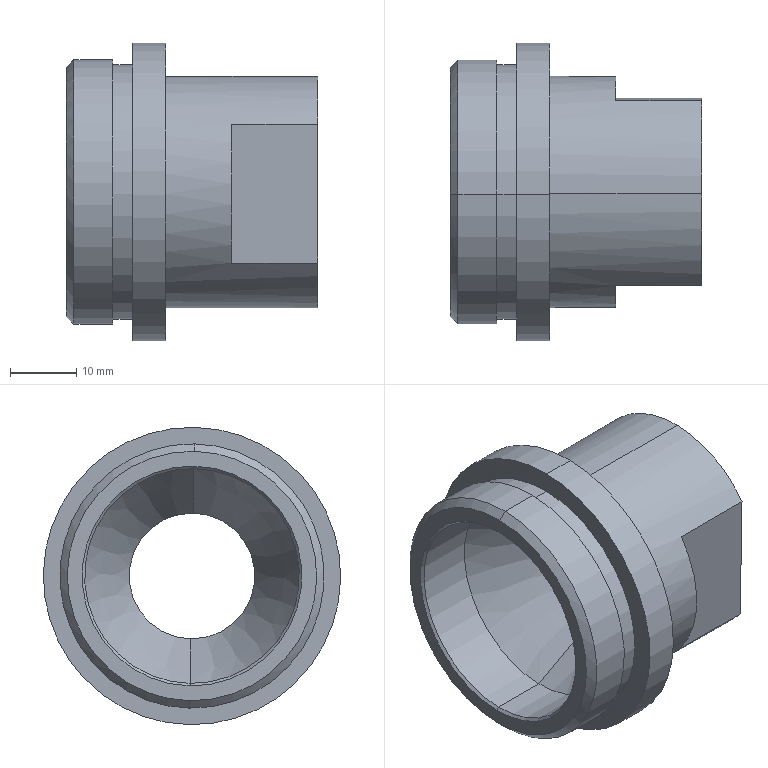Component | SolidWorks | 216InnerTubeAssembly-1_ValveGland-1 | 1 solid | 27 faces | box 38 x 45 x 45 mm | volume 22275 mm3 | cylinder 12 | plane 9 | cone 6 | commonest cylinder face diameters 40 x2 38.502 x2 45 x2 35 x2 19.03 x2 32.511 x2 | material Alloy Steel
build123d program:
from build123d import *

# Parameters (mm, degrees)
CUT_EXTRUDE1_DEPTH = 13


with BuildPart() as part:
    # Model → Revolve1 (revolve)
    with BuildSketch(Plane.XY, mode=Mode.PRIVATE) as revolve1_sk:
        Polygon((-37.447, 16.234), (-37.821, 16.608), (-37.821, 18.855), (-36.698, 19.979), (-30.821, 19.979), (-30.821, 19.23), (-27.821, 19.23), (-27.821, 22.479), (-22.821, 22.479), (-22.821, 17.479), (0.1786, 17.479), (0.1786, 9.494), (-16.821, 9.494), (-28.821, 16.234), align=None)
    revolve(revolve1_sk.sketch.rotate(Axis((1.198, -0.02131, 0), (-1, 0, 0)), 90), axis=Axis((1.198, -0.02131, 0), (-1, 0, 0)))

    # Sketch2 → Cut-Extrude1 (cut)
    with BuildSketch(Plane(origin=(0.1786, 0, 0), x_dir=(0, 0, -1), z_dir=(1, 0, 0))):
        with BuildLine():
            Line((-14.873, 13.979), (14.873, 13.979))
            ThreePointArc((14.873, 13.979), (0, 20.404), (-14.873, 13.979))
        make_face()
        with BuildLine():
            Line((-14.873, -14.021), (14.873, -14.021))
            ThreePointArc((14.873, -14.021), (0, -20.447), (-14.873, -14.021))
        make_face()
    extrude(amount=-CUT_EXTRUDE1_DEPTH, mode=Mode.SUBTRACT)


solid = part.part

# Placed as in the assembly
solid = solid.moved(Location((1191.249, 0.02131, 0.0003826), (1.029, 0, 0)))
STEP:
#1=COLOUR_RGB('',0.7922,0.8196,0.9333);
#2=FILL_AREA_STYLE_COLOUR('',#1);
#3=FILL_AREA_STYLE('',(#2));
#4=SURFACE_STYLE_FILL_AREA(#3);
#5=SURFACE_SIDE_STYLE('',(#4));
#6=SURFACE_STYLE_USAGE(.BOTH.,#5);
#7=PRESENTATION_STYLE_ASSIGNMENT((#6));
#8=CARTESIAN_POINT('',(45.425,-0.01149,0.6399));
#9=VERTEX_POINT('',#8);
#10=CARTESIAN_POINT('',(45.425,0.01149,-0.6399));
#11=VERTEX_POINT('',#10);
#12=CARTESIAN_POINT('',(45.425,-0.,0.));
#13=DIRECTION('',(1.,0.,-0.));
#14=DIRECTION('',(0.,0.01796,-0.9998));
#15=AXIS2_PLACEMENT_3D('',#12,#13,#14);
#16=CIRCLE('',#15,0.64);
#17=EDGE_CURVE('',#9,#11,#16,.T.);
#18=ORIENTED_EDGE('',*,*,#17,.T.);
#19=CARTESIAN_POINT('',(45.411,0.01176,-0.6546));
#20=VERTEX_POINT('',#19);
#21=CARTESIAN_POINT('',(45.411,0.01176,-0.6546));
#22=DIRECTION('',(-0.7071,0.0127,-0.707));
#23=VECTOR('',#22,39.37);
#24=LINE('',#21,#23);
#25=EDGE_CURVE('',#11,#20,#24,.T.);
#26=ORIENTED_EDGE('',*,*,#25,.T.);
#27=CARTESIAN_POINT('',(45.411,-0.01176,0.6546));
#28=VERTEX_POINT('',#27);
#29=CARTESIAN_POINT('',(45.411,-0.,0.));
#30=DIRECTION('',(1.,0.,-0.));
#31=DIRECTION('',(0.,0.01796,-0.9998));
#32=AXIS2_PLACEMENT_3D('',#29,#30,#31);
#33=CIRCLE('',#32,0.6547);
#34=EDGE_CURVE('',#28,#20,#33,.T.);
#35=ORIENTED_EDGE('',*,*,#34,.F.);
#36=CARTESIAN_POINT('',(45.411,-0.01176,0.6546));
#37=DIRECTION('',(-0.7071,-0.0127,0.707));
#38=VECTOR('',#37,39.37);
#39=LINE('',#36,#38);
#40=EDGE_CURVE('',#9,#28,#39,.T.);
#41=ORIENTED_EDGE('',*,*,#40,.F.);
#42=EDGE_LOOP('',(#18,#26,#35,#41));
#43=FACE_OUTER_BOUND('',#42,.T.);
#44=CARTESIAN_POINT('',(45.411,-0.,0.));
#45=DIRECTION('',(-1.,-0.,0.));
#46=DIRECTION('',(0.,-0.01796,0.9998));
#47=AXIS2_PLACEMENT_3D('',#44,#45,#46);
#48=CONICAL_SURFACE('',#47,0.6547,0.7854);
#49=ADVANCED_FACE('',(#43),#48,.F.);
#50=CARTESIAN_POINT('',(45.411,0.01334,-0.7431));
#51=VERTEX_POINT('',#50);
#52=CARTESIAN_POINT('',(45.411,-0.01334,0.7431));
#53=VERTEX_POINT('',#52);
#54=CARTESIAN_POINT('',(45.411,-0.,0.));
#55=DIRECTION('',(1.,0.,-0.));
#56=DIRECTION('',(0.,0.01796,-0.9998));
#57=AXIS2_PLACEMENT_3D('',#54,#55,#56);
#58=CIRCLE('',#57,0.7432);
#59=EDGE_CURVE('',#51,#53,#58,.T.);
#60=ORIENTED_EDGE('',*,*,#59,.T.);
#61=CARTESIAN_POINT('',(45.455,-0.01414,0.7873));
#62=VERTEX_POINT('',#61);
#63=CARTESIAN_POINT('',(45.455,-0.01414,0.7873));
#64=DIRECTION('',(0.7071,-0.0127,0.707));
#65=VECTOR('',#64,39.37);
#66=LINE('',#63,#65);
#67=EDGE_CURVE('',#53,#62,#66,.T.);
#68=ORIENTED_EDGE('',*,*,#67,.T.);
#69=CARTESIAN_POINT('',(45.455,0.01414,-0.7873));
#70=VERTEX_POINT('',#69);
#71=CARTESIAN_POINT('',(45.455,-0.,0.));
#72=DIRECTION('',(1.,0.,-0.));
#73=DIRECTION('',(0.,0.01796,-0.9998));
#74=AXIS2_PLACEMENT_3D('',#71,#72,#73);
#75=CIRCLE('',#74,0.7874);
#76=EDGE_CURVE('',#70,#62,#75,.T.);
#77=ORIENTED_EDGE('',*,*,#76,.F.);
#78=CARTESIAN_POINT('',(45.455,0.01414,-0.7873));
#79=DIRECTION('',(0.7071,0.0127,-0.707));
#80=VECTOR('',#79,39.37);
#81=LINE('',#78,#80);
#82=EDGE_CURVE('',#51,#70,#81,.T.);
#83=ORIENTED_EDGE('',*,*,#82,.F.);
#84=EDGE_LOOP('',(#60,#68,#77,#83));
#85=FACE_OUTER_BOUND('',#84,.T.);
#86=CARTESIAN_POINT('',(45.455,-0.,0.));
#87=DIRECTION('',(1.,0.,-0.));
#88=DIRECTION('',(0.,0.01796,-0.9998));
#89=AXIS2_PLACEMENT_3D('',#86,#87,#88);
#90=CONICAL_SURFACE('',#89,0.7874,0.7854);
#91=ADVANCED_FACE('',(#85),#90,.T.);
#92=ORIENTED_EDGE('',*,*,#76,.T.);
#93=CARTESIAN_POINT('',(45.686,-0.01414,0.7873));
#94=VERTEX_POINT('',#93);
#95=CARTESIAN_POINT('',(46.947,-0.01414,0.7873));
#96=DIRECTION('',(1.,0.,-0.));
#97=VECTOR('',#96,39.37);
#98=LINE('',#95,#97);
#99=EDGE_CURVE('',#62,#94,#98,.T.);
#100=ORIENTED_EDGE('',*,*,#99,.T.);
#101=CARTESIAN_POINT('',(45.686,0.01414,-0.7873));
#102=VERTEX_POINT('',#101);
#103=CARTESIAN_POINT('',(45.686,-0.,0.));
#104=DIRECTION('',(1.,0.,-0.));
#105=DIRECTION('',(0.,0.01796,-0.9998));
#106=AXIS2_PLACEMENT_3D('',#103,#104,#105);
#107=CIRCLE('',#106,0.7874);
#108=EDGE_CURVE('',#102,#94,#107,.T.);
#109=ORIENTED_EDGE('',*,*,#108,.F.);
#110=CARTESIAN_POINT('',(46.947,0.01414,-0.7873));
#111=DIRECTION('',(1.,0.,-0.));
#112=VECTOR('',#111,39.37);
#113=LINE('',#110,#112);
#114=EDGE_CURVE('',#70,#102,#113,.T.);
#115=ORIENTED_EDGE('',*,*,#114,.F.);
#116=EDGE_LOOP('',(#92,#100,#109,#115));
#117=FACE_OUTER_BOUND('',#116,.T.);
#118=CARTESIAN_POINT('',(46.947,-0.,0.));
#119=DIRECTION('',(1.,0.,-0.));
#120=DIRECTION('',(0.,0.01796,-0.9998));
#121=AXIS2_PLACEMENT_3D('',#118,#119,#120);
#122=CYLINDRICAL_SURFACE('',#121,0.7874);
#123=ADVANCED_FACE('',(#117),#122,.T.);
#124=CARTESIAN_POINT('',(45.686,0.01361,-0.7578));
#125=VERTEX_POINT('',#124);
#126=CARTESIAN_POINT('',(45.686,-0.01361,0.7578));
#127=VERTEX_POINT('',#126);
#128=CARTESIAN_POINT('',(45.686,-0.,0.));
#129=DIRECTION('',(1.,0.,-0.));
#130=DIRECTION('',(0.,0.01796,-0.9998));
#131=AXIS2_PLACEMENT_3D('',#128,#129,#130);
#132=CIRCLE('',#131,0.7579);
#133=EDGE_CURVE('',#125,#127,#132,.T.);
#134=ORIENTED_EDGE('',*,*,#133,.T.);
#135=CARTESIAN_POINT('',(45.804,-0.01361,0.7578));
#136=VERTEX_POINT('',#135);
#137=CARTESIAN_POINT('',(46.947,-0.01361,0.7578));
#138=DIRECTION('',(1.,0.,-0.));
#139=VECTOR('',#138,39.37);
#140=LINE('',#137,#139);
#141=EDGE_CURVE('',#127,#136,#140,.T.);
#142=ORIENTED_EDGE('',*,*,#141,.T.);
#143=CARTESIAN_POINT('',(45.804,0.01361,-0.7578));
#144=VERTEX_POINT('',#143);
#145=CARTESIAN_POINT('',(45.804,-0.,0.));
#146=DIRECTION('',(1.,0.,-0.));
#147=DIRECTION('',(0.,0.01796,-0.9998));
#148=AXIS2_PLACEMENT_3D('',#145,#146,#147);
#149=CIRCLE('',#148,0.7579);
#150=EDGE_CURVE('',#144,#136,#149,.T.);
#151=ORIENTED_EDGE('',*,*,#150,.F.);
#152=CARTESIAN_POINT('',(46.947,0.01361,-0.7578));
#153=DIRECTION('',(1.,0.,-0.));
#154=VECTOR('',#153,39.37);
#155=LINE('',#152,#154);
#156=EDGE_CURVE('',#125,#144,#155,.T.);
#157=ORIENTED_EDGE('',*,*,#156,.F.);
#158=EDGE_LOOP('',(#134,#142,#151,#157));
#159=FACE_OUTER_BOUND('',#158,.T.);
#160=CARTESIAN_POINT('',(46.947,-0.,0.));
#161=DIRECTION('',(1.,0.,-0.));
#162=DIRECTION('',(0.,0.01796,-0.9998));
#163=AXIS2_PLACEMENT_3D('',#160,#161,#162);
#164=CYLINDRICAL_SURFACE('',#163,0.7579);
#165=ADVANCED_FACE('',(#159),#164,.T.);
#166=CARTESIAN_POINT('',(45.804,0.01591,-0.8857));
#167=VERTEX_POINT('',#166);
#168=CARTESIAN_POINT('',(45.804,-0.01591,0.8857));
#169=VERTEX_POINT('',#168);
#170=CARTESIAN_POINT('',(45.804,-0.,0.));
#171=DIRECTION('',(1.,0.,-0.));
#172=DIRECTION('',(0.,0.01796,-0.9998));
#173=AXIS2_PLACEMENT_3D('',#170,#171,#172);
#174=CIRCLE('',#173,0.8858);
#175=EDGE_CURVE('',#167,#169,#174,.T.);
#176=ORIENTED_EDGE('',*,*,#175,.T.);
#177=CARTESIAN_POINT('',(46.001,-0.01591,0.8857));
#178=VERTEX_POINT('',#177);
#179=CARTESIAN_POINT('',(46.947,-0.01591,0.8857));
#180=DIRECTION('',(1.,0.,-0.));
#181=VECTOR('',#180,39.37);
#182=LINE('',#179,#181);
#183=EDGE_CURVE('',#169,#178,#182,.T.);
#184=ORIENTED_EDGE('',*,*,#183,.T.);
#185=CARTESIAN_POINT('',(46.001,0.01591,-0.8857));
#186=VERTEX_POINT('',#185);
#187=CARTESIAN_POINT('',(46.001,-0.,0.));
#188=DIRECTION('',(1.,0.,-0.));
#189=DIRECTION('',(0.,0.01796,-0.9998));
#190=AXIS2_PLACEMENT_3D('',#187,#188,#189);
#191=CIRCLE('',#190,0.8858);
#192=EDGE_CURVE('',#186,#178,#191,.T.);
#193=ORIENTED_EDGE('',*,*,#192,.F.);
#194=CARTESIAN_POINT('',(46.947,0.01591,-0.8857));
#195=DIRECTION('',(1.,0.,-0.));
#196=VECTOR('',#195,39.37);
#197=LINE('',#194,#196);
#198=EDGE_CURVE('',#167,#186,#197,.T.);
#199=ORIENTED_EDGE('',*,*,#198,.F.);
#200=EDGE_LOOP('',(#176,#184,#193,#199));
#201=FACE_OUTER_BOUND('',#200,.T.);
#202=CARTESIAN_POINT('',(46.947,-0.,0.));
#203=DIRECTION('',(1.,0.,-0.));
#204=DIRECTION('',(0.,0.01796,-0.9998));
#205=AXIS2_PLACEMENT_3D('',#202,#203,#204);
#206=CYLINDRICAL_SURFACE('',#205,0.8858);
#207=ADVANCED_FACE('',(#201),#206,.T.);
#208=CARTESIAN_POINT('',(46.001,0.01237,-0.6889));
#209=VERTEX_POINT('',#208);
#210=CARTESIAN_POINT('',(46.001,-0.01237,0.6889));
#211=VERTEX_POINT('',#210);
#212=CARTESIAN_POINT('',(46.001,-0.,0.));
#213=DIRECTION('',(1.,0.,-0.));
#214=DIRECTION('',(0.,0.01796,-0.9998));
#215=AXIS2_PLACEMENT_3D('',#212,#213,#214);
#216=CIRCLE('',#215,0.689);
#217=EDGE_CURVE('',#209,#211,#216,.T.);
#218=ORIENTED_EDGE('',*,*,#217,.T.);
#219=CARTESIAN_POINT('',(46.907,-0.01237,0.6889));
#220=VERTEX_POINT('',#219);
#221=CARTESIAN_POINT('',(46.947,-0.01237,0.6889));
#222=DIRECTION('',(1.,0.,-0.));
#223=VECTOR('',#222,39.37);
#224=LINE('',#221,#223);
#225=EDGE_CURVE('',#211,#220,#224,.T.);
#226=ORIENTED_EDGE('',*,*,#225,.T.);
#227=CARTESIAN_POINT('',(46.907,0.5437,0.4232));
#228=VERTEX_POINT('',#227);
#229=CARTESIAN_POINT('',(46.907,-0.,0.));
#230=DIRECTION('',(1.,0.,-0.));
#231=DIRECTION('',(0.,0.01796,-0.9998));
#232=AXIS2_PLACEMENT_3D('',#229,#230,#231);
#233=CIRCLE('',#232,0.689);
#234=EDGE_CURVE('',#228,#220,#233,.T.);
#235=ORIENTED_EDGE('',*,*,#234,.F.);
#236=CARTESIAN_POINT('',(46.395,0.5437,0.4232));
#237=VERTEX_POINT('',#236);
#238=CARTESIAN_POINT('',(46.947,0.5437,0.4232));
#239=DIRECTION('',(1.,0.,-0.));
#240=VECTOR('',#239,39.37);
#241=LINE('',#238,#240);
#242=EDGE_CURVE('',#237,#228,#241,.T.);
#243=ORIENTED_EDGE('',*,*,#242,.F.);
#244=CARTESIAN_POINT('',(46.395,0.5585,-0.4034));
#245=VERTEX_POINT('',#244);
#246=CARTESIAN_POINT('',(46.395,-0.,0.));
#247=DIRECTION('',(-1.,-0.,0.));
#248=DIRECTION('',(0.,0.01796,-0.9998));
#249=AXIS2_PLACEMENT_3D('',#246,#247,#248);
#250=CIRCLE('',#249,0.689);
#251=EDGE_CURVE('',#237,#245,#250,.T.);
#252=ORIENTED_EDGE('',*,*,#251,.T.);
#253=CARTESIAN_POINT('',(46.907,0.5585,-0.4034));
#254=VERTEX_POINT('',#253);
#255=CARTESIAN_POINT('',(46.947,0.5585,-0.4034));
#256=DIRECTION('',(-1.,-0.,0.));
#257=VECTOR('',#256,39.37);
#258=LINE('',#255,#257);
#259=EDGE_CURVE('',#254,#245,#258,.T.);
#260=ORIENTED_EDGE('',*,*,#259,.F.);
#261=CARTESIAN_POINT('',(46.907,0.01237,-0.6889));
#262=VERTEX_POINT('',#261);
#263=CARTESIAN_POINT('',(46.907,-0.,0.));
#264=DIRECTION('',(1.,0.,-0.));
#265=DIRECTION('',(0.,0.01796,-0.9998));
#266=AXIS2_PLACEMENT_3D('',#263,#264,#265);
#267=CIRCLE('',#266,0.689);
#268=EDGE_CURVE('',#262,#254,#267,.T.);
#269=ORIENTED_EDGE('',*,*,#268,.F.);
#270=CARTESIAN_POINT('',(46.947,0.01237,-0.6889));
#271=DIRECTION('',(1.,0.,-0.));
#272=VECTOR('',#271,39.37);
#273=LINE('',#270,#272);
#274=EDGE_CURVE('',#209,#262,#273,.T.);
#275=ORIENTED_EDGE('',*,*,#274,.F.);
#276=EDGE_LOOP('',(#218,#226,#235,#243,#252,#260,#269,#275));
#277=FACE_OUTER_BOUND('',#276,.T.);
#278=CARTESIAN_POINT('',(46.947,-0.,0.));
#279=DIRECTION('',(1.,0.,-0.));
#280=DIRECTION('',(0.,0.01796,-0.9998));
#281=AXIS2_PLACEMENT_3D('',#278,#279,#280);
#282=CYLINDRICAL_SURFACE('',#281,0.689);
#283=ADVANCED_FACE('',(#277),#282,.T.);
#284=CARTESIAN_POINT('',(46.237,-0.006726,0.3745));
#285=VERTEX_POINT('',#284);
#286=CARTESIAN_POINT('',(46.237,0.006726,-0.3745));
#287=VERTEX_POINT('',#286);
#288=CARTESIAN_POINT('',(46.237,-0.,0.));
#289=DIRECTION('',(1.,0.,-0.));
#290=DIRECTION('',(0.,0.01796,-0.9998));
#291=AXIS2_PLACEMENT_3D('',#288,#289,#290);
#292=CIRCLE('',#291,0.3746);
#293=EDGE_CURVE('',#285,#287,#292,.T.);
#294=ORIENTED_EDGE('',*,*,#293,.F.);
#295=CARTESIAN_POINT('',(46.907,-0.006726,0.3745));
#296=VERTEX_POINT('',#295);
#297=CARTESIAN_POINT('',(46.947,-0.006726,0.3745));
#298=DIRECTION('',(1.,0.,-0.));
#299=VECTOR('',#298,39.37);
#300=LINE('',#297,#299);
#301=EDGE_CURVE('',#285,#296,#300,.T.);
#302=ORIENTED_EDGE('',*,*,#301,.T.);
#303=CARTESIAN_POINT('',(46.907,0.006726,-0.3745));
#304=VERTEX_POINT('',#303);
#305=CARTESIAN_POINT('',(46.907,-0.,0.));
#306=DIRECTION('',(1.,0.,-0.));
#307=DIRECTION('',(0.,0.01796,-0.9998));
#308=AXIS2_PLACEMENT_3D('',#305,#306,#307);
#309=CIRCLE('',#308,0.3746);
#310=EDGE_CURVE('',#296,#304,#309,.T.);
#311=ORIENTED_EDGE('',*,*,#310,.T.);
#312=CARTESIAN_POINT('',(46.947,0.006726,-0.3745));
#313=DIRECTION('',(1.,0.,-0.));
#314=VECTOR('',#313,39.37);
#315=LINE('',#312,#314);
#316=EDGE_CURVE('',#287,#304,#315,.T.);
#317=ORIENTED_EDGE('',*,*,#316,.F.);
#318=EDGE_LOOP('',(#294,#302,#311,#317));
#319=FACE_OUTER_BOUND('',#318,.T.);
#320=CARTESIAN_POINT('',(46.947,-0.,0.));
#321=DIRECTION('',(1.,0.,-0.));
#322=DIRECTION('',(0.,0.01796,-0.9998));
#323=AXIS2_PLACEMENT_3D('',#320,#321,#322);
#324=CYLINDRICAL_SURFACE('',#323,0.3746);
#325=ADVANCED_FACE('',(#319),#324,.F.);
#326=ORIENTED_EDGE('',*,*,#293,.T.);
#327=CARTESIAN_POINT('',(45.765,0.01149,-0.6399));
#328=VERTEX_POINT('',#327);
#329=CARTESIAN_POINT('',(45.765,0.01149,-0.6399));
#330=DIRECTION('',(-0.8719,0.008794,-0.4897));
#331=VECTOR('',#330,39.37);
#332=LINE('',#329,#331);
#333=EDGE_CURVE('',#287,#328,#332,.T.);
#334=ORIENTED_EDGE('',*,*,#333,.T.);
#335=CARTESIAN_POINT('',(45.765,-0.01149,0.6399));
#336=VERTEX_POINT('',#335);
#337=CARTESIAN_POINT('',(45.765,-0.,0.));
#338=DIRECTION('',(1.,0.,-0.));
#339=DIRECTION('',(0.,0.01796,-0.9998));
#340=AXIS2_PLACEMENT_3D('',#337,#338,#339);
#341=CIRCLE('',#340,0.64);
#342=EDGE_CURVE('',#336,#328,#341,.T.);
#343=ORIENTED_EDGE('',*,*,#342,.F.);
#344=CARTESIAN_POINT('',(45.765,-0.01149,0.6399));
#345=DIRECTION('',(-0.8719,-0.008794,0.4897));
#346=VECTOR('',#345,39.37);
#347=LINE('',#344,#346);
#348=EDGE_CURVE('',#285,#336,#347,.T.);
#349=ORIENTED_EDGE('',*,*,#348,.F.);
#350=EDGE_LOOP('',(#326,#334,#343,#349));
#351=FACE_OUTER_BOUND('',#350,.T.);
#352=CARTESIAN_POINT('',(45.765,-0.,0.));
#353=DIRECTION('',(-1.,-0.,0.));
#354=DIRECTION('',(0.,-0.01796,0.9998));
#355=AXIS2_PLACEMENT_3D('',#352,#353,#354);
#356=CONICAL_SURFACE('',#355,0.64,0.5118);
#357=ADVANCED_FACE('',(#351),#356,.F.);
#358=ORIENTED_EDGE('',*,*,#17,.F.);
#359=CARTESIAN_POINT('',(46.947,-0.01149,0.6399));
#360=DIRECTION('',(1.,0.,-0.));
#361=VECTOR('',#360,39.37);
#362=LINE('',#359,#361);
#363=EDGE_CURVE('',#9,#336,#362,.T.);
#364=ORIENTED_EDGE('',*,*,#363,.T.);
#365=ORIENTED_EDGE('',*,*,#342,.T.);
#366=CARTESIAN_POINT('',(46.947,0.01149,-0.6399));
#367=DIRECTION('',(1.,0.,-0.));
#368=VECTOR('',#367,39.37);
#369=LINE('',#366,#368);
#370=EDGE_CURVE('',#11,#328,#369,.T.);
#371=ORIENTED_EDGE('',*,*,#370,.F.);
#372=EDGE_LOOP('',(#358,#364,#365,#371));
#373=FACE_OUTER_BOUND('',#372,.T.);
#374=CARTESIAN_POINT('',(46.947,-0.,0.));
#375=DIRECTION('',(1.,0.,-0.));
#376=DIRECTION('',(0.,0.01796,-0.9998));
#377=AXIS2_PLACEMENT_3D('',#374,#375,#376);
#378=CYLINDRICAL_SURFACE('',#377,0.64);
#379=ADVANCED_FACE('',(#373),#378,.F.);
#380=ORIENTED_EDGE('',*,*,#363,.F.);
#381=CARTESIAN_POINT('',(45.425,-0.,0.));
#382=DIRECTION('',(1.,0.,-0.));
#383=DIRECTION('',(0.,0.01796,-0.9998));
#384=AXIS2_PLACEMENT_3D('',#381,#382,#383);
#385=CIRCLE('',#384,0.64);
#386=EDGE_CURVE('',#11,#9,#385,.T.);
#387=ORIENTED_EDGE('',*,*,#386,.F.);
#388=ORIENTED_EDGE('',*,*,#370,.T.);
#389=CARTESIAN_POINT('',(45.765,-0.,0.));
#390=DIRECTION('',(1.,0.,-0.));
#391=DIRECTION('',(0.,0.01796,-0.9998));
#392=AXIS2_PLACEMENT_3D('',#389,#390,#391);
#393=CIRCLE('',#392,0.64);
#394=EDGE_CURVE('',#328,#336,#393,.T.);
#395=ORIENTED_EDGE('',*,*,#394,.T.);
#396=EDGE_LOOP('',(#380,#387,#388,#395));
#397=FACE_OUTER_BOUND('',#396,.T.);
#398=CARTESIAN_POINT('',(46.947,-0.,0.));
#399=DIRECTION('',(1.,0.,-0.));
#400=DIRECTION('',(0.,0.01796,-0.9998));
#401=AXIS2_PLACEMENT_3D('',#398,#399,#400);
#402=CYLINDRICAL_SURFACE('',#401,0.64);
#403=ADVANCED_FACE('',(#397),#402,.F.);
#404=ORIENTED_EDGE('',*,*,#333,.F.);
#405=CARTESIAN_POINT('',(46.237,-0.,0.));
#406=DIRECTION('',(1.,0.,-0.));
#407=DIRECTION('',(0.,0.01796,-0.9998));
#408=AXIS2_PLACEMENT_3D('',#405,#406,#407);
#409=CIRCLE('',#408,0.3746);
#410=EDGE_CURVE('',#287,#285,#409,.T.);
#411=ORIENTED_EDGE('',*,*,#410,.T.);
#412=ORIENTED_EDGE('',*,*,#348,.T.);
#413=ORIENTED_EDGE('',*,*,#394,.F.);
#414=EDGE_LOOP('',(#404,#411,#412,#413));
#415=FACE_OUTER_BOUND('',#414,.T.);
#416=CARTESIAN_POINT('',(45.765,-0.,0.));
#417=DIRECTION('',(-1.,-0.,0.));
#418=DIRECTION('',(0.,-0.01796,0.9998));
#419=AXIS2_PLACEMENT_3D('',#416,#417,#418);
#420=CONICAL_SURFACE('',#419,0.64,0.5118);
#421=ADVANCED_FACE('',(#415),#420,.F.);
#422=ORIENTED_EDGE('',*,*,#301,.F.);
#423=ORIENTED_EDGE('',*,*,#410,.F.);
#424=ORIENTED_EDGE('',*,*,#316,.T.);
#425=CARTESIAN_POINT('',(46.907,-0.,0.));
#426=DIRECTION('',(1.,0.,-0.));
#427=DIRECTION('',(0.,0.01796,-0.9998));
#428=AXIS2_PLACEMENT_3D('',#425,#426,#427);
#429=CIRCLE('',#428,0.3746);
#430=EDGE_CURVE('',#304,#296,#429,.T.);
#431=ORIENTED_EDGE('',*,*,#430,.T.);
#432=EDGE_LOOP('',(#422,#423,#424,#431));
#433=FACE_OUTER_BOUND('',#432,.T.);
#434=CARTESIAN_POINT('',(46.947,-0.,0.));
#435=DIRECTION('',(1.,0.,-0.));
#436=DIRECTION('',(0.,0.01796,-0.9998));
#437=AXIS2_PLACEMENT_3D('',#434,#435,#436);
#438=CYLINDRICAL_SURFACE('',#437,0.3746);
#439=ADVANCED_FACE('',(#433),#438,.F.);
#440=CARTESIAN_POINT('',(46.907,0.5406,0.5954));
#441=DIRECTION('',(-0.,0.01796,-0.9998));
#442=VECTOR('',#441,39.37);
#443=LINE('',#440,#442);
#444=EDGE_CURVE('',#228,#254,#443,.T.);
#445=ORIENTED_EDGE('',*,*,#444,.F.);
#446=ORIENTED_EDGE('',*,*,#234,.T.);
#447=CARTESIAN_POINT('',(46.907,-0.5585,0.4034));
#448=VERTEX_POINT('',#447);
#449=CARTESIAN_POINT('',(46.907,-0.,0.));
#450=DIRECTION('',(1.,0.,-0.));
#451=DIRECTION('',(0.,0.01796,-0.9998));
#452=AXIS2_PLACEMENT_3D('',#449,#450,#451);
#453=CIRCLE('',#452,0.689);
#454=EDGE_CURVE('',#220,#448,#453,.T.);
#455=ORIENTED_EDGE('',*,*,#454,.T.);
#456=CARTESIAN_POINT('',(46.907,-0.5437,-0.4232));
#457=VERTEX_POINT('',#456);
#458=CARTESIAN_POINT('',(46.907,-0.5616,0.5756));
#459=DIRECTION('',(0.,-0.01796,0.9998));
#460=VECTOR('',#459,39.37);
#461=LINE('',#458,#460);
#462=EDGE_CURVE('',#457,#448,#461,.T.);
#463=ORIENTED_EDGE('',*,*,#462,.F.);
#464=CARTESIAN_POINT('',(46.907,-0.,0.));
#465=DIRECTION('',(1.,0.,-0.));
#466=DIRECTION('',(0.,0.01796,-0.9998));
#467=AXIS2_PLACEMENT_3D('',#464,#465,#466);
#468=CIRCLE('',#467,0.689);
#469=EDGE_CURVE('',#457,#262,#468,.T.);
#470=ORIENTED_EDGE('',*,*,#469,.T.);
#471=ORIENTED_EDGE('',*,*,#268,.T.);
#472=EDGE_LOOP('',(#445,#446,#455,#463,#470,#471));
#473=FACE_OUTER_BOUND('',#472,.T.);
#474=ORIENTED_EDGE('',*,*,#430,.F.);
#475=ORIENTED_EDGE('',*,*,#310,.F.);
#476=EDGE_LOOP('',(#474,#475));
#477=FACE_BOUND('',#476,.T.);
#478=CARTESIAN_POINT('',(46.907,0.3745,0.006726));
#479=DIRECTION('',(1.,0.,-0.));
#480=DIRECTION('',(-0.,0.01796,-0.9998));
#481=AXIS2_PLACEMENT_3D('',#478,#479,#480);
#482=PLANE('',#481);
#483=ADVANCED_FACE('',(#473,#477),#482,.T.);
#484=ORIENTED_EDGE('',*,*,#225,.F.);
#485=CARTESIAN_POINT('',(46.001,-0.,0.));
#486=DIRECTION('',(1.,0.,-0.));
#487=DIRECTION('',(0.,0.01796,-0.9998));
#488=AXIS2_PLACEMENT_3D('',#485,#486,#487);
#489=CIRCLE('',#488,0.689);
#490=EDGE_CURVE('',#211,#209,#489,.T.);
#491=ORIENTED_EDGE('',*,*,#490,.T.);
#492=ORIENTED_EDGE('',*,*,#274,.T.);
#493=ORIENTED_EDGE('',*,*,#469,.F.);
#494=CARTESIAN_POINT('',(46.395,-0.5437,-0.4232));
#495=VERTEX_POINT('',#494);
#496=CARTESIAN_POINT('',(46.947,-0.5437,-0.4232));
#497=DIRECTION('',(1.,0.,-0.));
#498=VECTOR('',#497,39.37);
#499=LINE('',#496,#498);
#500=EDGE_CURVE('',#495,#457,#499,.T.);
#501=ORIENTED_EDGE('',*,*,#500,.F.);
#502=CARTESIAN_POINT('',(46.395,-0.5585,0.4034));
#503=VERTEX_POINT('',#502);
#504=CARTESIAN_POINT('',(46.395,-0.,0.));
#505=DIRECTION('',(-1.,-0.,0.));
#506=DIRECTION('',(0.,0.01796,-0.9998));
#507=AXIS2_PLACEMENT_3D('',#504,#505,#506);
#508=CIRCLE('',#507,0.689);
#509=EDGE_CURVE('',#495,#503,#508,.T.);
#510=ORIENTED_EDGE('',*,*,#509,.T.);
#511=CARTESIAN_POINT('',(46.947,-0.5585,0.4034));
#512=DIRECTION('',(-1.,-0.,0.));
#513=VECTOR('',#512,39.37);
#514=LINE('',#511,#513);
#515=EDGE_CURVE('',#448,#503,#514,.T.);
#516=ORIENTED_EDGE('',*,*,#515,.F.);
#517=ORIENTED_EDGE('',*,*,#454,.F.);
#518=EDGE_LOOP('',(#484,#491,#492,#493,#501,#510,#516,#517));
#519=FACE_OUTER_BOUND('',#518,.T.);
#520=CARTESIAN_POINT('',(46.947,-0.,0.));
#521=DIRECTION('',(1.,0.,-0.));
#522=DIRECTION('',(0.,0.01796,-0.9998));
#523=AXIS2_PLACEMENT_3D('',#520,#521,#522);
#524=CYLINDRICAL_SURFACE('',#523,0.689);
#525=ADVANCED_FACE('',(#519),#524,.T.);
#526=ORIENTED_EDGE('',*,*,#192,.T.);
#527=CARTESIAN_POINT('',(46.001,-0.,0.));
#528=DIRECTION('',(1.,0.,-0.));
#529=DIRECTION('',(0.,0.01796,-0.9998));
#530=AXIS2_PLACEMENT_3D('',#527,#528,#529);
#531=CIRCLE('',#530,0.8858);
#532=EDGE_CURVE('',#178,#186,#531,.T.);
#533=ORIENTED_EDGE('',*,*,#532,.T.);
#534=EDGE_LOOP('',(#526,#533));
#535=FACE_OUTER_BOUND('',#534,.T.);
#536=ORIENTED_EDGE('',*,*,#217,.F.);
#537=ORIENTED_EDGE('',*,*,#490,.F.);
#538=EDGE_LOOP('',(#536,#537));
#539=FACE_BOUND('',#538,.T.);
#540=CARTESIAN_POINT('',(46.001,0.6889,0.01237));
#541=DIRECTION('',(1.,0.,-0.));
#542=DIRECTION('',(-0.,0.01796,-0.9998));
#543=AXIS2_PLACEMENT_3D('',#540,#541,#542);
#544=PLANE('',#543);
#545=ADVANCED_FACE('',(#535,#539),#544,.T.);
#546=ORIENTED_EDGE('',*,*,#183,.F.);
#547=CARTESIAN_POINT('',(45.804,-0.,0.));
#548=DIRECTION('',(1.,0.,-0.));
#549=DIRECTION('',(0.,0.01796,-0.9998));
#550=AXIS2_PLACEMENT_3D('',#547,#548,#549);
#551=CIRCLE('',#550,0.8858);
#552=EDGE_CURVE('',#169,#167,#551,.T.);
#553=ORIENTED_EDGE('',*,*,#552,.T.);
#554=ORIENTED_EDGE('',*,*,#198,.T.);
#555=ORIENTED_EDGE('',*,*,#532,.F.);
#556=EDGE_LOOP('',(#546,#553,#554,#555));
#557=FACE_OUTER_BOUND('',#556,.T.);
#558=CARTESIAN_POINT('',(46.947,-0.,0.));
#559=DIRECTION('',(1.,0.,-0.));
#560=DIRECTION('',(0.,0.01796,-0.9998));
#561=AXIS2_PLACEMENT_3D('',#558,#559,#560);
#562=CYLINDRICAL_SURFACE('',#561,0.8858);
#563=ADVANCED_FACE('',(#557),#562,.T.);
#564=ORIENTED_EDGE('',*,*,#150,.T.);
#565=CARTESIAN_POINT('',(45.804,-0.,0.));
#566=DIRECTION('',(1.,0.,-0.));
#567=DIRECTION('',(0.,0.01796,-0.9998));
#568=AXIS2_PLACEMENT_3D('',#565,#566,#567);
#569=CIRCLE('',#568,0.7579);
#570=EDGE_CURVE('',#136,#144,#569,.T.);
#571=ORIENTED_EDGE('',*,*,#570,.T.);
#572=EDGE_LOOP('',(#564,#571));
#573=FACE_BOUND('',#572,.T.);
#574=ORIENTED_EDGE('',*,*,#175,.F.);
#575=ORIENTED_EDGE('',*,*,#552,.F.);
#576=EDGE_LOOP('',(#574,#575));
#577=FACE_OUTER_BOUND('',#576,.T.);
#578=CARTESIAN_POINT('',(45.804,0.7578,0.01361));
#579=DIRECTION('',(-1.,-0.,0.));
#580=DIRECTION('',(0.,-0.01796,0.9998));
#581=AXIS2_PLACEMENT_3D('',#578,#579,#580);
#582=PLANE('',#581);
#583=ADVANCED_FACE('',(#573,#577),#582,.T.);
#584=ORIENTED_EDGE('',*,*,#141,.F.);
#585=CARTESIAN_POINT('',(45.686,-0.,0.));
#586=DIRECTION('',(1.,0.,-0.));
#587=DIRECTION('',(0.,0.01796,-0.9998));
#588=AXIS2_PLACEMENT_3D('',#585,#586,#587);
#589=CIRCLE('',#588,0.7579);
#590=EDGE_CURVE('',#127,#125,#589,.T.);
#591=ORIENTED_EDGE('',*,*,#590,.T.);
#592=ORIENTED_EDGE('',*,*,#156,.T.);
#593=ORIENTED_EDGE('',*,*,#570,.F.);
#594=EDGE_LOOP('',(#584,#591,#592,#593));
#595=FACE_OUTER_BOUND('',#594,.T.);
#596=CARTESIAN_POINT('',(46.947,-0.,0.));
#597=DIRECTION('',(1.,0.,-0.));
#598=DIRECTION('',(0.,0.01796,-0.9998));
#599=AXIS2_PLACEMENT_3D('',#596,#597,#598);
#600=CYLINDRICAL_SURFACE('',#599,0.7579);
#601=ADVANCED_FACE('',(#595),#600,.T.);
#602=ORIENTED_EDGE('',*,*,#108,.T.);
#603=CARTESIAN_POINT('',(45.686,-0.,0.));
#604=DIRECTION('',(1.,0.,-0.));
#605=DIRECTION('',(0.,0.01796,-0.9998));
#606=AXIS2_PLACEMENT_3D('',#603,#604,#605);
#607=CIRCLE('',#606,0.7874);
#608=EDGE_CURVE('',#94,#102,#607,.T.);
#609=ORIENTED_EDGE('',*,*,#608,.T.);
#610=EDGE_LOOP('',(#602,#609));
#611=FACE_OUTER_BOUND('',#610,.T.);
#612=ORIENTED_EDGE('',*,*,#133,.F.);
#613=ORIENTED_EDGE('',*,*,#590,.F.);
#614=EDGE_LOOP('',(#612,#613));
#615=FACE_BOUND('',#614,.T.);
#616=CARTESIAN_POINT('',(45.686,0.7873,0.01414));
#617=DIRECTION('',(1.,0.,-0.));
#618=DIRECTION('',(-0.,0.01796,-0.9998));
#619=AXIS2_PLACEMENT_3D('',#616,#617,#618);
#620=PLANE('',#619);
#621=ADVANCED_FACE('',(#611,#615),#620,.T.);
#622=ORIENTED_EDGE('',*,*,#99,.F.);
#623=CARTESIAN_POINT('',(45.455,-0.,0.));
#624=DIRECTION('',(1.,0.,-0.));
#625=DIRECTION('',(0.,0.01796,-0.9998));
#626=AXIS2_PLACEMENT_3D('',#623,#624,#625);
#627=CIRCLE('',#626,0.7874);
#628=EDGE_CURVE('',#62,#70,#627,.T.);
#629=ORIENTED_EDGE('',*,*,#628,.T.);
#630=ORIENTED_EDGE('',*,*,#114,.T.);
#631=ORIENTED_EDGE('',*,*,#608,.F.);
#632=EDGE_LOOP('',(#622,#629,#630,#631));
#633=FACE_OUTER_BOUND('',#632,.T.);
#634=CARTESIAN_POINT('',(46.947,-0.,0.));
#635=DIRECTION('',(1.,0.,-0.));
#636=DIRECTION('',(0.,0.01796,-0.9998));
#637=AXIS2_PLACEMENT_3D('',#634,#635,#636);
#638=CYLINDRICAL_SURFACE('',#637,0.7874);
#639=ADVANCED_FACE('',(#633),#638,.T.);
#640=ORIENTED_EDGE('',*,*,#67,.F.);
#641=CARTESIAN_POINT('',(45.411,-0.,0.));
#642=DIRECTION('',(1.,0.,-0.));
#643=DIRECTION('',(0.,0.01796,-0.9998));
#644=AXIS2_PLACEMENT_3D('',#641,#642,#643);
#645=CIRCLE('',#644,0.7432);
#646=EDGE_CURVE('',#53,#51,#645,.T.);
#647=ORIENTED_EDGE('',*,*,#646,.T.);
#648=ORIENTED_EDGE('',*,*,#82,.T.);
#649=ORIENTED_EDGE('',*,*,#628,.F.);
#650=EDGE_LOOP('',(#640,#647,#648,#649));
#651=FACE_OUTER_BOUND('',#650,.T.);
#652=CARTESIAN_POINT('',(45.455,-0.,0.));
#653=DIRECTION('',(1.,0.,-0.));
#654=DIRECTION('',(0.,0.01796,-0.9998));
#655=AXIS2_PLACEMENT_3D('',#652,#653,#654);
#656=CONICAL_SURFACE('',#655,0.7874,0.7854);
#657=ADVANCED_FACE('',(#651),#656,.T.);
#658=ORIENTED_EDGE('',*,*,#34,.T.);
#659=CARTESIAN_POINT('',(45.411,-0.,0.));
#660=DIRECTION('',(1.,0.,-0.));
#661=DIRECTION('',(0.,0.01796,-0.9998));
#662=AXIS2_PLACEMENT_3D('',#659,#660,#661);
#663=CIRCLE('',#662,0.6547);
#664=EDGE_CURVE('',#20,#28,#663,.T.);
#665=ORIENTED_EDGE('',*,*,#664,.T.);
#666=EDGE_LOOP('',(#658,#665));
#667=FACE_BOUND('',#666,.T.);
#668=ORIENTED_EDGE('',*,*,#59,.F.);
#669=ORIENTED_EDGE('',*,*,#646,.F.);
#670=EDGE_LOOP('',(#668,#669));
#671=FACE_OUTER_BOUND('',#670,.T.);
#672=CARTESIAN_POINT('',(45.411,0.7431,0.01334));
#673=DIRECTION('',(-1.,-0.,0.));
#674=DIRECTION('',(0.,-0.01796,0.9998));
#675=AXIS2_PLACEMENT_3D('',#672,#673,#674);
#676=PLANE('',#675);
#677=ADVANCED_FACE('',(#667,#671),#676,.T.);
#678=ORIENTED_EDGE('',*,*,#25,.F.);
#679=ORIENTED_EDGE('',*,*,#386,.T.);
#680=ORIENTED_EDGE('',*,*,#40,.T.);
#681=ORIENTED_EDGE('',*,*,#664,.F.);
#682=EDGE_LOOP('',(#678,#679,#680,#681));
#683=FACE_OUTER_BOUND('',#682,.T.);
#684=CARTESIAN_POINT('',(45.411,-0.,0.));
#685=DIRECTION('',(-1.,-0.,0.));
#686=DIRECTION('',(0.,-0.01796,0.9998));
#687=AXIS2_PLACEMENT_3D('',#684,#685,#686);
#688=CONICAL_SURFACE('',#687,0.6547,0.7854);
#689=ADVANCED_FACE('',(#683),#688,.F.);
#690=ORIENTED_EDGE('',*,*,#515,.T.);
#691=CARTESIAN_POINT('',(46.395,-0.5616,0.5756));
#692=DIRECTION('',(0.,-0.01796,0.9998));
#693=VECTOR('',#692,39.37);
#694=LINE('',#691,#693);
#695=EDGE_CURVE('',#495,#503,#694,.T.);
#696=ORIENTED_EDGE('',*,*,#695,.F.);
#697=ORIENTED_EDGE('',*,*,#500,.T.);
#698=ORIENTED_EDGE('',*,*,#462,.T.);
#699=EDGE_LOOP('',(#690,#696,#697,#698));
#700=FACE_OUTER_BOUND('',#699,.T.);
#701=CARTESIAN_POINT('',(46.395,-0.5616,0.5756));
#702=DIRECTION('',(0.,0.9998,0.01796));
#703=DIRECTION('',(0.,-0.01796,0.9998));
#704=AXIS2_PLACEMENT_3D('',#701,#702,#703);
#705=PLANE('',#704);
#706=ADVANCED_FACE('',(#700),#705,.F.);
#707=ORIENTED_EDGE('',*,*,#695,.T.);
#708=ORIENTED_EDGE('',*,*,#509,.F.);
#709=EDGE_LOOP('',(#707,#708));
#710=FACE_OUTER_BOUND('',#709,.T.);
#711=CARTESIAN_POINT('',(46.395,-0.,0.));
#712=DIRECTION('',(1.,0.,-0.));
#713=DIRECTION('',(-0.,0.01796,-0.9998));
#714=AXIS2_PLACEMENT_3D('',#711,#712,#713);
#715=PLANE('',#714);
#716=ADVANCED_FACE('',(#710),#715,.T.);
#717=ORIENTED_EDGE('',*,*,#259,.T.);
#718=CARTESIAN_POINT('',(46.395,0.5406,0.5954));
#719=DIRECTION('',(-0.,0.01796,-0.9998));
#720=VECTOR('',#719,39.37);
#721=LINE('',#718,#720);
#722=EDGE_CURVE('',#237,#245,#721,.T.);
#723=ORIENTED_EDGE('',*,*,#722,.F.);
#724=ORIENTED_EDGE('',*,*,#242,.T.);
#725=ORIENTED_EDGE('',*,*,#444,.T.);
#726=EDGE_LOOP('',(#717,#723,#724,#725));
#727=FACE_OUTER_BOUND('',#726,.T.);
#728=CARTESIAN_POINT('',(46.395,0.5406,0.5954));
#729=DIRECTION('',(-0.,-0.9998,-0.01796));
#730=DIRECTION('',(-0.,0.01796,-0.9998));
#731=AXIS2_PLACEMENT_3D('',#728,#729,#730);
#732=PLANE('',#731);
#733=ADVANCED_FACE('',(#727),#732,.F.);
#734=ORIENTED_EDGE('',*,*,#722,.T.);
#735=ORIENTED_EDGE('',*,*,#251,.F.);
#736=EDGE_LOOP('',(#734,#735));
#737=FACE_OUTER_BOUND('',#736,.T.);
#738=CARTESIAN_POINT('',(46.395,-0.,0.));
#739=DIRECTION('',(1.,0.,-0.));
#740=DIRECTION('',(-0.,0.01796,-0.9998));
#741=AXIS2_PLACEMENT_3D('',#738,#739,#740);
#742=PLANE('',#741);
#743=ADVANCED_FACE('',(#737),#742,.T.);
#744=CLOSED_SHELL('',(#49,#91,#123,#165,#207,#283,#325,#357,#379,#403,#421,#439,#483,#525,#545,#563,#583,#601,#621,#639,#657,#677,#689,#706,#716,#733,#743));
#745=MANIFOLD_SOLID_BREP('',#744);
#746=STYLED_ITEM('',(#7),#745);
#747=(LENGTH_UNIT()NAMED_UNIT(*)SI_UNIT($,.METRE.));
#748=LENGTH_MEASURE_WITH_UNIT(LENGTH_MEASURE(0.0254),#747);
#749=DIMENSIONAL_EXPONENTS(1.,0.,0.,0.,0.,0.,0.);
#750=(CONVERSION_BASED_UNIT('',#748)LENGTH_UNIT()NAMED_UNIT(#749));
#751=UNCERTAINTY_MEASURE_WITH_UNIT(LENGTH_MEASURE(0.00001),#750,'','');
#752=(NAMED_UNIT(*)PLANE_ANGLE_UNIT()SI_UNIT($,.RADIAN.));
#753=(NAMED_UNIT(*)SI_UNIT($,.STERADIAN.)SOLID_ANGLE_UNIT());
#754=(GEOMETRIC_REPRESENTATION_CONTEXT(3)GLOBAL_UNCERTAINTY_ASSIGNED_CONTEXT((#751))GLOBAL_UNIT_ASSIGNED_CONTEXT((#750,#752,#753))REPRESENTATION_CONTEXT('',''));
#755=MECHANICAL_DESIGN_GEOMETRIC_PRESENTATION_REPRESENTATION('',(#746),#754);
#756=CARTESIAN_POINT('',(0.,0.,0.));
#757=DIRECTION('',(0.,0.,1.));
#758=DIRECTION('',(1.,0.,0.));
#759=AXIS2_PLACEMENT_3D('',#756,#757,#758);
#760=(LENGTH_UNIT()NAMED_UNIT(*)SI_UNIT($,.METRE.));
#761=LENGTH_MEASURE_WITH_UNIT(LENGTH_MEASURE(0.0254),#760);
#762=DIMENSIONAL_EXPONENTS(1.,0.,0.,0.,0.,0.,0.);
#763=(CONVERSION_BASED_UNIT('',#761)LENGTH_UNIT()NAMED_UNIT(#762));
#764=UNCERTAINTY_MEASURE_WITH_UNIT(LENGTH_MEASURE(0.00001),#763,'','');
#765=(NAMED_UNIT(*)PLANE_ANGLE_UNIT()SI_UNIT($,.RADIAN.));
#766=(NAMED_UNIT(*)SI_UNIT($,.STERADIAN.)SOLID_ANGLE_UNIT());
#767=(GEOMETRIC_REPRESENTATION_CONTEXT(3)GLOBAL_UNCERTAINTY_ASSIGNED_CONTEXT((#764))GLOBAL_UNIT_ASSIGNED_CONTEXT((#763,#765,#766))REPRESENTATION_CONTEXT('',''));
#768=ADVANCED_BREP_SHAPE_REPRESENTATION('',(#745,#759),#767);
#769=PRESENTATION_LAYER_ASSIGNMENT('','',(#746));